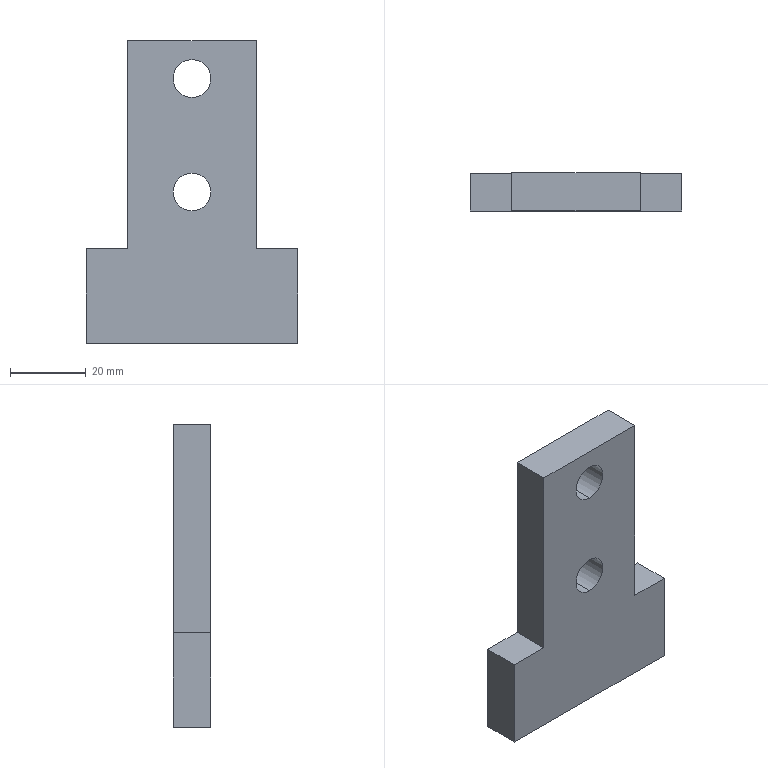Component | SolidWorks | 03-1 | 1 solid | 14 faces | box 56 x 10 x 80 mm | volume 31129 mm3 | plane 10 | cylinder 4 | commonest cylinder face diameters 10 x4
build123d program:
from build123d import *

# Parameters (mm, degrees)
SKETCH1_W           = 56
SKETCH1_H           = 80
SKETCH1_R           = 5
BOSS_EXTRUDE1_DEPTH = 5
SKETCH2_W           = 11
SKETCH2_H           = 55
CUT_EXTRUDE1_DEPTH  = 50.84


with BuildPart() as part:
    # Sketch1 → Boss-Extrude1 (new, symmetric)
    with BuildSketch(Plane(origin=(0, 0, 0), x_dir=(1, 0, 0), z_dir=(0, 1, 0))):
        Rectangle(SKETCH1_W, SKETCH1_H)
        with Locations(Location((0, -30, 0), (0, 0, 270))):
            Circle(SKETCH1_R, mode=Mode.SUBTRACT)
        with Locations(Location((0, 0, 0), (0, 0, 270))):
            Circle(SKETCH1_R, mode=Mode.SUBTRACT)
    extrude(amount=BOSS_EXTRUDE1_DEPTH, both=True)

    # Sketch2 → Cut-Extrude1 (cut, through all)
    with BuildSketch(Plane(origin=(0, 5, 0), x_dir=(1, 0, 0), z_dir=(0, 1, 0))):
        with Locations((-22.5, -12.5)):
            Rectangle(SKETCH2_W, SKETCH2_H)
        with Locations((22.5, -12.5)):
            Rectangle(SKETCH2_W, SKETCH2_H)
    extrude(amount=-CUT_EXTRUDE1_DEPTH, mode=Mode.SUBTRACT)


solid = part.part

# Placed as in the assembly
solid = solid.moved(Location((-42, 156.3, 86), (0, 0, 0)))
STEP:
#1=COLOUR_RGB('',0.7922,0.8196,0.9333);
#2=FILL_AREA_STYLE_COLOUR('',#1);
#3=FILL_AREA_STYLE('',(#2));
#4=SURFACE_STYLE_FILL_AREA(#3);
#5=SURFACE_SIDE_STYLE('',(#4));
#6=SURFACE_STYLE_USAGE(.BOTH.,#5);
#7=PRESENTATION_STYLE_ASSIGNMENT((#6));
#8=CARTESIAN_POINT('',(-1.654,6.35,3.189));
#9=VERTEX_POINT('',#8);
#10=CARTESIAN_POINT('',(-1.654,6.35,3.583));
#11=VERTEX_POINT('',#10);
#12=CARTESIAN_POINT('',(-1.654,6.35,3.386));
#13=DIRECTION('',(0.,1.,0.));
#14=DIRECTION('',(0.,0.,1.));
#15=AXIS2_PLACEMENT_3D('',#12,#13,#14);
#16=CIRCLE('',#15,0.1969);
#17=EDGE_CURVE('',#9,#11,#16,.T.);
#18=ORIENTED_EDGE('',*,*,#17,.T.);
#19=CARTESIAN_POINT('',(-1.654,5.957,3.583));
#20=VERTEX_POINT('',#19);
#21=CARTESIAN_POINT('',(-1.654,6.35,3.583));
#22=DIRECTION('',(0.,-1.,0.));
#23=VECTOR('',#22,39.37);
#24=LINE('',#21,#23);
#25=EDGE_CURVE('',#11,#20,#24,.T.);
#26=ORIENTED_EDGE('',*,*,#25,.T.);
#27=CARTESIAN_POINT('',(-1.654,5.957,3.189));
#28=VERTEX_POINT('',#27);
#29=CARTESIAN_POINT('',(-1.654,5.957,3.386));
#30=DIRECTION('',(0.,1.,0.));
#31=DIRECTION('',(0.,0.,1.));
#32=AXIS2_PLACEMENT_3D('',#29,#30,#31);
#33=CIRCLE('',#32,0.1969);
#34=EDGE_CURVE('',#28,#20,#33,.T.);
#35=ORIENTED_EDGE('',*,*,#34,.F.);
#36=CARTESIAN_POINT('',(-1.654,6.35,3.189));
#37=DIRECTION('',(0.,-1.,0.));
#38=VECTOR('',#37,39.37);
#39=LINE('',#36,#38);
#40=EDGE_CURVE('',#9,#28,#39,.T.);
#41=ORIENTED_EDGE('',*,*,#40,.F.);
#42=EDGE_LOOP('',(#18,#26,#35,#41));
#43=FACE_OUTER_BOUND('',#42,.T.);
#44=CARTESIAN_POINT('',(-1.654,6.35,3.386));
#45=DIRECTION('',(0.,-1.,0.));
#46=DIRECTION('',(0.,0.,-1.));
#47=AXIS2_PLACEMENT_3D('',#44,#45,#46);
#48=CYLINDRICAL_SURFACE('',#47,0.1969);
#49=ADVANCED_FACE('',(#43),#48,.F.);
#50=CARTESIAN_POINT('',(-1.654,6.35,4.37));
#51=VERTEX_POINT('',#50);
#52=CARTESIAN_POINT('',(-1.654,6.35,4.764));
#53=VERTEX_POINT('',#52);
#54=CARTESIAN_POINT('',(-1.654,6.35,4.567));
#55=DIRECTION('',(0.,1.,0.));
#56=DIRECTION('',(0.,0.,1.));
#57=AXIS2_PLACEMENT_3D('',#54,#55,#56);
#58=CIRCLE('',#57,0.1969);
#59=EDGE_CURVE('',#51,#53,#58,.T.);
#60=ORIENTED_EDGE('',*,*,#59,.T.);
#61=CARTESIAN_POINT('',(-1.654,5.957,4.764));
#62=VERTEX_POINT('',#61);
#63=CARTESIAN_POINT('',(-1.654,6.35,4.764));
#64=DIRECTION('',(0.,-1.,0.));
#65=VECTOR('',#64,39.37);
#66=LINE('',#63,#65);
#67=EDGE_CURVE('',#53,#62,#66,.T.);
#68=ORIENTED_EDGE('',*,*,#67,.T.);
#69=CARTESIAN_POINT('',(-1.654,5.957,4.37));
#70=VERTEX_POINT('',#69);
#71=CARTESIAN_POINT('',(-1.654,5.957,4.567));
#72=DIRECTION('',(0.,1.,0.));
#73=DIRECTION('',(0.,0.,1.));
#74=AXIS2_PLACEMENT_3D('',#71,#72,#73);
#75=CIRCLE('',#74,0.1969);
#76=EDGE_CURVE('',#70,#62,#75,.T.);
#77=ORIENTED_EDGE('',*,*,#76,.F.);
#78=CARTESIAN_POINT('',(-1.654,6.35,4.37));
#79=DIRECTION('',(0.,-1.,0.));
#80=VECTOR('',#79,39.37);
#81=LINE('',#78,#80);
#82=EDGE_CURVE('',#51,#70,#81,.T.);
#83=ORIENTED_EDGE('',*,*,#82,.F.);
#84=EDGE_LOOP('',(#60,#68,#77,#83));
#85=FACE_OUTER_BOUND('',#84,.T.);
#86=CARTESIAN_POINT('',(-1.654,6.35,4.567));
#87=DIRECTION('',(0.,-1.,0.));
#88=DIRECTION('',(0.,0.,-1.));
#89=AXIS2_PLACEMENT_3D('',#86,#87,#88);
#90=CYLINDRICAL_SURFACE('',#89,0.1969);
#91=ADVANCED_FACE('',(#85),#90,.F.);
#92=CARTESIAN_POINT('',(-2.323,6.35,4.961));
#93=VERTEX_POINT('',#92);
#94=CARTESIAN_POINT('',(-0.9843,6.35,4.961));
#95=VERTEX_POINT('',#94);
#96=CARTESIAN_POINT('',(-2.756,6.35,4.961));
#97=DIRECTION('',(1.,0.,0.));
#98=VECTOR('',#97,39.37);
#99=LINE('',#96,#98);
#100=EDGE_CURVE('',#93,#95,#99,.T.);
#101=ORIENTED_EDGE('',*,*,#100,.T.);
#102=CARTESIAN_POINT('',(-0.9843,6.35,2.795));
#103=VERTEX_POINT('',#102);
#104=CARTESIAN_POINT('',(-0.9843,6.35,4.961));
#105=DIRECTION('',(0.,0.,1.));
#106=VECTOR('',#105,39.37);
#107=LINE('',#104,#106);
#108=EDGE_CURVE('',#103,#95,#107,.T.);
#109=ORIENTED_EDGE('',*,*,#108,.F.);
#110=CARTESIAN_POINT('',(-0.5512,6.35,2.795));
#111=VERTEX_POINT('',#110);
#112=CARTESIAN_POINT('',(-0.5512,6.35,2.795));
#113=DIRECTION('',(-1.,0.,0.));
#114=VECTOR('',#113,39.37);
#115=LINE('',#112,#114);
#116=EDGE_CURVE('',#111,#103,#115,.T.);
#117=ORIENTED_EDGE('',*,*,#116,.F.);
#118=CARTESIAN_POINT('',(-0.5512,6.35,1.811));
#119=VERTEX_POINT('',#118);
#120=CARTESIAN_POINT('',(-0.5512,6.35,4.961));
#121=DIRECTION('',(0.,0.,-1.));
#122=VECTOR('',#121,39.37);
#123=LINE('',#120,#122);
#124=EDGE_CURVE('',#111,#119,#123,.T.);
#125=ORIENTED_EDGE('',*,*,#124,.T.);
#126=CARTESIAN_POINT('',(-2.756,6.35,1.811));
#127=VERTEX_POINT('',#126);
#128=CARTESIAN_POINT('',(-2.756,6.35,1.811));
#129=DIRECTION('',(-1.,0.,0.));
#130=VECTOR('',#129,39.37);
#131=LINE('',#128,#130);
#132=EDGE_CURVE('',#119,#127,#131,.T.);
#133=ORIENTED_EDGE('',*,*,#132,.T.);
#134=CARTESIAN_POINT('',(-2.756,6.35,2.795));
#135=VERTEX_POINT('',#134);
#136=CARTESIAN_POINT('',(-2.756,6.35,4.961));
#137=DIRECTION('',(0.,0.,1.));
#138=VECTOR('',#137,39.37);
#139=LINE('',#136,#138);
#140=EDGE_CURVE('',#127,#135,#139,.T.);
#141=ORIENTED_EDGE('',*,*,#140,.T.);
#142=CARTESIAN_POINT('',(-2.323,6.35,2.795));
#143=VERTEX_POINT('',#142);
#144=CARTESIAN_POINT('',(-2.756,6.35,2.795));
#145=DIRECTION('',(-1.,0.,0.));
#146=VECTOR('',#145,39.37);
#147=LINE('',#144,#146);
#148=EDGE_CURVE('',#143,#135,#147,.T.);
#149=ORIENTED_EDGE('',*,*,#148,.F.);
#150=CARTESIAN_POINT('',(-2.323,6.35,4.961));
#151=DIRECTION('',(0.,0.,-1.));
#152=VECTOR('',#151,39.37);
#153=LINE('',#150,#152);
#154=EDGE_CURVE('',#93,#143,#153,.T.);
#155=ORIENTED_EDGE('',*,*,#154,.F.);
#156=EDGE_LOOP('',(#101,#109,#117,#125,#133,#141,#149,#155));
#157=FACE_OUTER_BOUND('',#156,.T.);
#158=ORIENTED_EDGE('',*,*,#59,.F.);
#159=CARTESIAN_POINT('',(-1.654,6.35,4.567));
#160=DIRECTION('',(0.,1.,0.));
#161=DIRECTION('',(0.,0.,1.));
#162=AXIS2_PLACEMENT_3D('',#159,#160,#161);
#163=CIRCLE('',#162,0.1969);
#164=EDGE_CURVE('',#53,#51,#163,.T.);
#165=ORIENTED_EDGE('',*,*,#164,.F.);
#166=EDGE_LOOP('',(#158,#165));
#167=FACE_BOUND('',#166,.T.);
#168=ORIENTED_EDGE('',*,*,#17,.F.);
#169=CARTESIAN_POINT('',(-1.654,6.35,3.386));
#170=DIRECTION('',(0.,1.,0.));
#171=DIRECTION('',(0.,0.,1.));
#172=AXIS2_PLACEMENT_3D('',#169,#170,#171);
#173=CIRCLE('',#172,0.1969);
#174=EDGE_CURVE('',#11,#9,#173,.T.);
#175=ORIENTED_EDGE('',*,*,#174,.F.);
#176=EDGE_LOOP('',(#168,#175));
#177=FACE_BOUND('',#176,.T.);
#178=CARTESIAN_POINT('',(-1.654,6.35,3.386));
#179=DIRECTION('',(0.,-1.,0.));
#180=DIRECTION('',(0.,0.,-1.));
#181=AXIS2_PLACEMENT_3D('',#178,#179,#180);
#182=PLANE('',#181);
#183=ADVANCED_FACE('',(#157,#167,#177),#182,.F.);
#184=CARTESIAN_POINT('',(-0.9843,5.957,2.795));
#185=VERTEX_POINT('',#184);
#186=CARTESIAN_POINT('',(-0.9843,5.957,4.961));
#187=VERTEX_POINT('',#186);
#188=CARTESIAN_POINT('',(-0.9843,5.957,4.961));
#189=DIRECTION('',(0.,0.,1.));
#190=VECTOR('',#189,39.37);
#191=LINE('',#188,#190);
#192=EDGE_CURVE('',#185,#187,#191,.T.);
#193=ORIENTED_EDGE('',*,*,#192,.T.);
#194=CARTESIAN_POINT('',(-2.323,5.957,4.961));
#195=VERTEX_POINT('',#194);
#196=CARTESIAN_POINT('',(-2.756,5.957,4.961));
#197=DIRECTION('',(1.,0.,0.));
#198=VECTOR('',#197,39.37);
#199=LINE('',#196,#198);
#200=EDGE_CURVE('',#195,#187,#199,.T.);
#201=ORIENTED_EDGE('',*,*,#200,.F.);
#202=CARTESIAN_POINT('',(-2.323,5.957,2.795));
#203=VERTEX_POINT('',#202);
#204=CARTESIAN_POINT('',(-2.323,5.957,4.961));
#205=DIRECTION('',(0.,0.,-1.));
#206=VECTOR('',#205,39.37);
#207=LINE('',#204,#206);
#208=EDGE_CURVE('',#195,#203,#207,.T.);
#209=ORIENTED_EDGE('',*,*,#208,.T.);
#210=CARTESIAN_POINT('',(-2.756,5.957,2.795));
#211=VERTEX_POINT('',#210);
#212=CARTESIAN_POINT('',(-2.756,5.957,2.795));
#213=DIRECTION('',(-1.,0.,0.));
#214=VECTOR('',#213,39.37);
#215=LINE('',#212,#214);
#216=EDGE_CURVE('',#203,#211,#215,.T.);
#217=ORIENTED_EDGE('',*,*,#216,.T.);
#218=CARTESIAN_POINT('',(-2.756,5.957,1.811));
#219=VERTEX_POINT('',#218);
#220=CARTESIAN_POINT('',(-2.756,5.957,4.961));
#221=DIRECTION('',(0.,0.,1.));
#222=VECTOR('',#221,39.37);
#223=LINE('',#220,#222);
#224=EDGE_CURVE('',#219,#211,#223,.T.);
#225=ORIENTED_EDGE('',*,*,#224,.F.);
#226=CARTESIAN_POINT('',(-0.5512,5.957,1.811));
#227=VERTEX_POINT('',#226);
#228=CARTESIAN_POINT('',(-2.756,5.957,1.811));
#229=DIRECTION('',(-1.,0.,0.));
#230=VECTOR('',#229,39.37);
#231=LINE('',#228,#230);
#232=EDGE_CURVE('',#227,#219,#231,.T.);
#233=ORIENTED_EDGE('',*,*,#232,.F.);
#234=CARTESIAN_POINT('',(-0.5512,5.957,2.795));
#235=VERTEX_POINT('',#234);
#236=CARTESIAN_POINT('',(-0.5512,5.957,4.961));
#237=DIRECTION('',(0.,0.,-1.));
#238=VECTOR('',#237,39.37);
#239=LINE('',#236,#238);
#240=EDGE_CURVE('',#235,#227,#239,.T.);
#241=ORIENTED_EDGE('',*,*,#240,.F.);
#242=CARTESIAN_POINT('',(-0.5512,5.957,2.795));
#243=DIRECTION('',(-1.,0.,0.));
#244=VECTOR('',#243,39.37);
#245=LINE('',#242,#244);
#246=EDGE_CURVE('',#235,#185,#245,.T.);
#247=ORIENTED_EDGE('',*,*,#246,.T.);
#248=EDGE_LOOP('',(#193,#201,#209,#217,#225,#233,#241,#247));
#249=FACE_OUTER_BOUND('',#248,.T.);
#250=ORIENTED_EDGE('',*,*,#76,.T.);
#251=CARTESIAN_POINT('',(-1.654,5.957,4.567));
#252=DIRECTION('',(0.,1.,0.));
#253=DIRECTION('',(0.,0.,1.));
#254=AXIS2_PLACEMENT_3D('',#251,#252,#253);
#255=CIRCLE('',#254,0.1969);
#256=EDGE_CURVE('',#62,#70,#255,.T.);
#257=ORIENTED_EDGE('',*,*,#256,.T.);
#258=EDGE_LOOP('',(#250,#257));
#259=FACE_BOUND('',#258,.T.);
#260=ORIENTED_EDGE('',*,*,#34,.T.);
#261=CARTESIAN_POINT('',(-1.654,5.957,3.386));
#262=DIRECTION('',(0.,1.,0.));
#263=DIRECTION('',(0.,0.,1.));
#264=AXIS2_PLACEMENT_3D('',#261,#262,#263);
#265=CIRCLE('',#264,0.1969);
#266=EDGE_CURVE('',#20,#28,#265,.T.);
#267=ORIENTED_EDGE('',*,*,#266,.T.);
#268=EDGE_LOOP('',(#260,#267));
#269=FACE_BOUND('',#268,.T.);
#270=CARTESIAN_POINT('',(-1.654,5.957,3.386));
#271=DIRECTION('',(0.,-1.,0.));
#272=DIRECTION('',(0.,0.,-1.));
#273=AXIS2_PLACEMENT_3D('',#270,#271,#272);
#274=PLANE('',#273);
#275=ADVANCED_FACE('',(#249,#259,#269),#274,.T.);
#276=ORIENTED_EDGE('',*,*,#124,.F.);
#277=CARTESIAN_POINT('',(-0.5512,5.957,2.795));
#278=DIRECTION('',(0.,1.,0.));
#279=VECTOR('',#278,39.37);
#280=LINE('',#277,#279);
#281=EDGE_CURVE('',#235,#111,#280,.T.);
#282=ORIENTED_EDGE('',*,*,#281,.F.);
#283=ORIENTED_EDGE('',*,*,#240,.T.);
#284=CARTESIAN_POINT('',(-0.5512,6.35,1.811));
#285=DIRECTION('',(0.,-1.,0.));
#286=VECTOR('',#285,39.37);
#287=LINE('',#284,#286);
#288=EDGE_CURVE('',#119,#227,#287,.T.);
#289=ORIENTED_EDGE('',*,*,#288,.F.);
#290=EDGE_LOOP('',(#276,#282,#283,#289));
#291=FACE_OUTER_BOUND('',#290,.T.);
#292=CARTESIAN_POINT('',(-0.5512,6.35,4.961));
#293=DIRECTION('',(-1.,0.,-0.));
#294=DIRECTION('',(-0.,0.,1.));
#295=AXIS2_PLACEMENT_3D('',#292,#293,#294);
#296=PLANE('',#295);
#297=ADVANCED_FACE('',(#291),#296,.F.);
#298=ORIENTED_EDGE('',*,*,#232,.T.);
#299=CARTESIAN_POINT('',(-2.756,6.35,1.811));
#300=DIRECTION('',(0.,-1.,0.));
#301=VECTOR('',#300,39.37);
#302=LINE('',#299,#301);
#303=EDGE_CURVE('',#127,#219,#302,.T.);
#304=ORIENTED_EDGE('',*,*,#303,.F.);
#305=ORIENTED_EDGE('',*,*,#132,.F.);
#306=ORIENTED_EDGE('',*,*,#288,.T.);
#307=EDGE_LOOP('',(#298,#304,#305,#306));
#308=FACE_OUTER_BOUND('',#307,.T.);
#309=CARTESIAN_POINT('',(-2.756,6.35,1.811));
#310=DIRECTION('',(0.,0.,1.));
#311=DIRECTION('',(1.,0.,0.));
#312=AXIS2_PLACEMENT_3D('',#309,#310,#311);
#313=PLANE('',#312);
#314=ADVANCED_FACE('',(#308),#313,.F.);
#315=ORIENTED_EDGE('',*,*,#224,.T.);
#316=CARTESIAN_POINT('',(-2.756,5.957,2.795));
#317=DIRECTION('',(0.,1.,0.));
#318=VECTOR('',#317,39.37);
#319=LINE('',#316,#318);
#320=EDGE_CURVE('',#211,#135,#319,.T.);
#321=ORIENTED_EDGE('',*,*,#320,.T.);
#322=ORIENTED_EDGE('',*,*,#140,.F.);
#323=ORIENTED_EDGE('',*,*,#303,.T.);
#324=EDGE_LOOP('',(#315,#321,#322,#323));
#325=FACE_OUTER_BOUND('',#324,.T.);
#326=CARTESIAN_POINT('',(-2.756,6.35,4.961));
#327=DIRECTION('',(1.,0.,0.));
#328=DIRECTION('',(0.,0.,-1.));
#329=AXIS2_PLACEMENT_3D('',#326,#327,#328);
#330=PLANE('',#329);
#331=ADVANCED_FACE('',(#325),#330,.F.);
#332=ORIENTED_EDGE('',*,*,#200,.T.);
#333=CARTESIAN_POINT('',(-0.9843,5.957,4.961));
#334=DIRECTION('',(0.,1.,0.));
#335=VECTOR('',#334,39.37);
#336=LINE('',#333,#335);
#337=EDGE_CURVE('',#187,#95,#336,.T.);
#338=ORIENTED_EDGE('',*,*,#337,.T.);
#339=ORIENTED_EDGE('',*,*,#100,.F.);
#340=CARTESIAN_POINT('',(-2.323,5.957,4.961));
#341=DIRECTION('',(0.,1.,0.));
#342=VECTOR('',#341,39.37);
#343=LINE('',#340,#342);
#344=EDGE_CURVE('',#195,#93,#343,.T.);
#345=ORIENTED_EDGE('',*,*,#344,.F.);
#346=EDGE_LOOP('',(#332,#338,#339,#345));
#347=FACE_OUTER_BOUND('',#346,.T.);
#348=CARTESIAN_POINT('',(-2.756,6.35,4.961));
#349=DIRECTION('',(0.,0.,-1.));
#350=DIRECTION('',(-1.,0.,-0.));
#351=AXIS2_PLACEMENT_3D('',#348,#349,#350);
#352=PLANE('',#351);
#353=ADVANCED_FACE('',(#347),#352,.F.);
#354=ORIENTED_EDGE('',*,*,#67,.F.);
#355=ORIENTED_EDGE('',*,*,#164,.T.);
#356=ORIENTED_EDGE('',*,*,#82,.T.);
#357=ORIENTED_EDGE('',*,*,#256,.F.);
#358=EDGE_LOOP('',(#354,#355,#356,#357));
#359=FACE_OUTER_BOUND('',#358,.T.);
#360=CARTESIAN_POINT('',(-1.654,6.35,4.567));
#361=DIRECTION('',(0.,-1.,0.));
#362=DIRECTION('',(0.,0.,-1.));
#363=AXIS2_PLACEMENT_3D('',#360,#361,#362);
#364=CYLINDRICAL_SURFACE('',#363,0.1969);
#365=ADVANCED_FACE('',(#359),#364,.F.);
#366=ORIENTED_EDGE('',*,*,#25,.F.);
#367=ORIENTED_EDGE('',*,*,#174,.T.);
#368=ORIENTED_EDGE('',*,*,#40,.T.);
#369=ORIENTED_EDGE('',*,*,#266,.F.);
#370=EDGE_LOOP('',(#366,#367,#368,#369));
#371=FACE_OUTER_BOUND('',#370,.T.);
#372=CARTESIAN_POINT('',(-1.654,6.35,3.386));
#373=DIRECTION('',(0.,-1.,0.));
#374=DIRECTION('',(0.,0.,-1.));
#375=AXIS2_PLACEMENT_3D('',#372,#373,#374);
#376=CYLINDRICAL_SURFACE('',#375,0.1969);
#377=ADVANCED_FACE('',(#371),#376,.F.);
#378=ORIENTED_EDGE('',*,*,#148,.T.);
#379=ORIENTED_EDGE('',*,*,#320,.F.);
#380=ORIENTED_EDGE('',*,*,#216,.F.);
#381=CARTESIAN_POINT('',(-2.323,5.957,2.795));
#382=DIRECTION('',(0.,1.,0.));
#383=VECTOR('',#382,39.37);
#384=LINE('',#381,#383);
#385=EDGE_CURVE('',#203,#143,#384,.T.);
#386=ORIENTED_EDGE('',*,*,#385,.T.);
#387=EDGE_LOOP('',(#378,#379,#380,#386));
#388=FACE_OUTER_BOUND('',#387,.T.);
#389=CARTESIAN_POINT('',(-2.756,5.957,2.795));
#390=DIRECTION('',(0.,0.,-1.));
#391=DIRECTION('',(-1.,0.,0.));
#392=AXIS2_PLACEMENT_3D('',#389,#390,#391);
#393=PLANE('',#392);
#394=ADVANCED_FACE('',(#388),#393,.F.);
#395=ORIENTED_EDGE('',*,*,#154,.T.);
#396=ORIENTED_EDGE('',*,*,#385,.F.);
#397=ORIENTED_EDGE('',*,*,#208,.F.);
#398=ORIENTED_EDGE('',*,*,#344,.T.);
#399=EDGE_LOOP('',(#395,#396,#397,#398));
#400=FACE_OUTER_BOUND('',#399,.T.);
#401=CARTESIAN_POINT('',(-2.323,5.957,4.961));
#402=DIRECTION('',(1.,0.,0.));
#403=DIRECTION('',(0.,0.,-1.));
#404=AXIS2_PLACEMENT_3D('',#401,#402,#403);
#405=PLANE('',#404);
#406=ADVANCED_FACE('',(#400),#405,.F.);
#407=ORIENTED_EDGE('',*,*,#108,.T.);
#408=ORIENTED_EDGE('',*,*,#337,.F.);
#409=ORIENTED_EDGE('',*,*,#192,.F.);
#410=CARTESIAN_POINT('',(-0.9843,5.957,2.795));
#411=DIRECTION('',(0.,1.,0.));
#412=VECTOR('',#411,39.37);
#413=LINE('',#410,#412);
#414=EDGE_CURVE('',#185,#103,#413,.T.);
#415=ORIENTED_EDGE('',*,*,#414,.T.);
#416=EDGE_LOOP('',(#407,#408,#409,#415));
#417=FACE_OUTER_BOUND('',#416,.T.);
#418=CARTESIAN_POINT('',(-0.9843,5.957,4.961));
#419=DIRECTION('',(-1.,0.,0.));
#420=DIRECTION('',(0.,0.,1.));
#421=AXIS2_PLACEMENT_3D('',#418,#419,#420);
#422=PLANE('',#421);
#423=ADVANCED_FACE('',(#417),#422,.F.);
#424=ORIENTED_EDGE('',*,*,#116,.T.);
#425=ORIENTED_EDGE('',*,*,#414,.F.);
#426=ORIENTED_EDGE('',*,*,#246,.F.);
#427=ORIENTED_EDGE('',*,*,#281,.T.);
#428=EDGE_LOOP('',(#424,#425,#426,#427));
#429=FACE_OUTER_BOUND('',#428,.T.);
#430=CARTESIAN_POINT('',(-0.5512,5.957,2.795));
#431=DIRECTION('',(0.,0.,-1.));
#432=DIRECTION('',(-1.,0.,0.));
#433=AXIS2_PLACEMENT_3D('',#430,#431,#432);
#434=PLANE('',#433);
#435=ADVANCED_FACE('',(#429),#434,.F.);
#436=CLOSED_SHELL('',(#49,#91,#183,#275,#297,#314,#331,#353,#365,#377,#394,#406,#423,#435));
#437=MANIFOLD_SOLID_BREP('',#436);
#438=STYLED_ITEM('',(#7),#437);
#439=(LENGTH_UNIT()NAMED_UNIT(*)SI_UNIT($,.METRE.));
#440=LENGTH_MEASURE_WITH_UNIT(LENGTH_MEASURE(0.0254),#439);
#441=DIMENSIONAL_EXPONENTS(1.,0.,0.,0.,0.,0.,0.);
#442=(CONVERSION_BASED_UNIT('',#440)LENGTH_UNIT()NAMED_UNIT(#441));
#443=UNCERTAINTY_MEASURE_WITH_UNIT(LENGTH_MEASURE(0.00001),#442,'','');
#444=(NAMED_UNIT(*)PLANE_ANGLE_UNIT()SI_UNIT($,.RADIAN.));
#445=(NAMED_UNIT(*)SI_UNIT($,.STERADIAN.)SOLID_ANGLE_UNIT());
#446=(GEOMETRIC_REPRESENTATION_CONTEXT(3)GLOBAL_UNCERTAINTY_ASSIGNED_CONTEXT((#443))GLOBAL_UNIT_ASSIGNED_CONTEXT((#442,#444,#445))REPRESENTATION_CONTEXT('',''));
#447=MECHANICAL_DESIGN_GEOMETRIC_PRESENTATION_REPRESENTATION('',(#438),#446);
#448=PRESENTATION_LAYER_ASSIGNMENT('','',(#438));
#449=CARTESIAN_POINT('',(0.,0.,0.));
#450=DIRECTION('',(0.,0.,1.));
#451=DIRECTION('',(1.,0.,0.));
#452=AXIS2_PLACEMENT_3D('',#449,#450,#451);
#453=(LENGTH_UNIT()NAMED_UNIT(*)SI_UNIT($,.METRE.));
#454=LENGTH_MEASURE_WITH_UNIT(LENGTH_MEASURE(0.0254),#453);
#455=DIMENSIONAL_EXPONENTS(1.,0.,0.,0.,0.,0.,0.);
#456=(CONVERSION_BASED_UNIT('',#454)LENGTH_UNIT()NAMED_UNIT(#455));
#457=UNCERTAINTY_MEASURE_WITH_UNIT(LENGTH_MEASURE(0.00001),#456,'','');
#458=(NAMED_UNIT(*)PLANE_ANGLE_UNIT()SI_UNIT($,.RADIAN.));
#459=(NAMED_UNIT(*)SI_UNIT($,.STERADIAN.)SOLID_ANGLE_UNIT());
#460=(GEOMETRIC_REPRESENTATION_CONTEXT(3)GLOBAL_UNCERTAINTY_ASSIGNED_CONTEXT((#457))GLOBAL_UNIT_ASSIGNED_CONTEXT((#456,#458,#459))REPRESENTATION_CONTEXT('',''));
#461=ADVANCED_BREP_SHAPE_REPRESENTATION('',(#437,#452),#460);